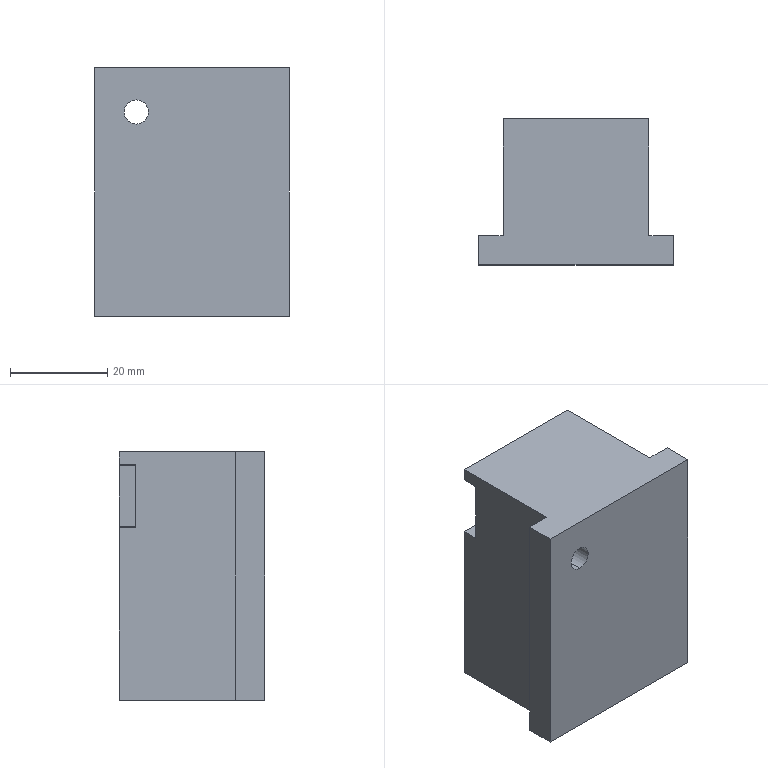Component | SolidWorks | PusherSeat-1 | 1 solid | 23 faces | box 40 x 30 x 51.1 mm | volume 47655 mm3 | plane 14 | cylinder 7 | cone 2 | commonest cylinder face diameters 0.5 x3 5 x2 2.5 x2 | material 201 Annealed Stainless Steel (SS)
build123d program:
from build123d import *

# Parameters (mm, degrees)
SKETCH1_W                 = 40
SKETCH1_H                 = 30
EXTRUDE1_DEPTH            = 30
M3X0_5_TAPPED_HOLE2_D     = 2.5
M3X0_5_TAPPED_HOLE2_DEPTH = 7.5
M3X0_5_TAPPED_HOLE2_TIP   = 0.7511
SKETCH15_W                = 30
SKETCH15_H                = 30
CUT_EXTRUDE5_DEPTH        = 1.2
SKETCH17_3_W              = 6
SKETCH17_3_H              = 5
BOSS_EXTRUDE5_DEPTH       = 30
SKETCH17_3_2_W            = 6
SKETCH17_3_2_H            = 5
BOSS_EXTRUDE6_DEPTH       = 38.8
SKETCH23_W                = 30
SKETCH23_H                = 10
BOSS_EXTRUDE7_DEPTH       = 5
BOSS_EXTRUDE8_DEPTH       = 12.3
SKETCH30_W                = 13
SKETCH30_H                = 19
CUT_EXTRUDE6_DEPTH        = 3.4
SKETCH31_W                = 7.3
SKETCH31_H                = 10
BOSS_EXTRUDE9_DEPTH       = 26.6
SKETCH32_W                = 2.6
SKETCH32_H                = 10
BOSS_EXTRUDE10_DEPTH      = 3.4
SKETCH33_R                = 2.5
CUT_EXTRUDE7_DEPTH        = 68.407
SKETCH34_W                = 6
SKETCH34_H                = 5
BOSS_EXTRUDE11_DEPTH      = 21.1
SKETCH35_R                = 0.25
CUT_EXTRUDE8_DEPTH        = 3.4


with BuildPart() as part:
    # Sketch1 → Extrude1 (new body)
    with BuildSketch(Plane.XY):
        with Locations((20, 15)):
            Rectangle(SKETCH1_W, SKETCH1_H)
    extrude(amount=EXTRUDE1_DEPTH)

    # M3x0.5 Tapped Hole2
    with Locations(Plane.ZY):
        with Locations((15, 15)):
            Hole(M3X0_5_TAPPED_HOLE2_D / 2, depth=M3X0_5_TAPPED_HOLE2_DEPTH)
            with Locations((0, 0, -(M3X0_5_TAPPED_HOLE2_DEPTH + M3X0_5_TAPPED_HOLE2_TIP / 2))):  # 118° drill point
                Cone(0, M3X0_5_TAPPED_HOLE2_D / 2, M3X0_5_TAPPED_HOLE2_TIP, mode=Mode.SUBTRACT)

    # Sketch15 → Cut-Extrude5 (cut)
    with BuildSketch(Plane(origin=(40, 0, 0), x_dir=(0, 0, -1), z_dir=(1, 0, 0))):
        with Locations((-15, 15)):
            Rectangle(SKETCH15_W, SKETCH15_H)
    extrude(amount=-CUT_EXTRUDE5_DEPTH, mode=Mode.SUBTRACT)

    # Sketch17_3 → Boss-Extrude5 (add)
    with BuildSketch(Plane.ZY):
        with Locations((3, -2.5)):
            Rectangle(SKETCH17_3_W, SKETCH17_3_H)
    extrude(amount=-BOSS_EXTRUDE5_DEPTH)

    # Sketch17_3 2 → Boss-Extrude6 (add)
    with BuildSketch(Plane.ZY):
        with Locations((3, 32.5)):
            Rectangle(SKETCH17_3_2_W, SKETCH17_3_2_H)
    extrude(amount=-BOSS_EXTRUDE6_DEPTH)

    # Sketch23 → Boss-Extrude7 (add)
    with BuildSketch(Plane(origin=(38.8, 0, 0), x_dir=(0, 0, -1), z_dir=(1, 0, 0))):
        with Locations((-15, 5)):
            Rectangle(SKETCH23_W, SKETCH23_H)
    extrude(amount=BOSS_EXTRUDE7_DEPTH)

    # Sketch24 → Boss-Extrude8 (add)
    with BuildSketch(Plane(origin=(38.8, 0, 0), x_dir=(0, 0, -1), z_dir=(1, 0, 0))):
        Polygon((-30, 10), (-30, 30), (-6, 30), (-6, 35), (0, 35), (0, 10), align=None)
    extrude(amount=BOSS_EXTRUDE8_DEPTH)

    # Sketch30 → Cut-Extrude6 (cut)
    with BuildSketch(Plane.XY.offset(30)):
        with Locations((42, 9.5)):
            Rectangle(SKETCH30_W, SKETCH30_H)
    extrude(amount=-CUT_EXTRUDE6_DEPTH, mode=Mode.SUBTRACT)

    # Sketch31 → Boss-Extrude9 (add)
    with BuildSketch(Plane(origin=(0, 0, 0), x_dir=(-1, 0, 0), z_dir=(0, 0, -1))):
        with Locations((-47.45, 5)):
            Rectangle(SKETCH31_W, SKETCH31_H)
    extrude(amount=-BOSS_EXTRUDE9_DEPTH)

    # Sketch32 → Boss-Extrude10 (add)
    with BuildSketch(Plane.XY.offset(26.6)):
        with Locations((49.8, 5)):
            Rectangle(SKETCH32_W, SKETCH32_H)
    extrude(amount=BOSS_EXTRUDE10_DEPTH)

    # Sketch33 → Cut-Extrude7 (cut, through all)
    with BuildSketch(Plane.XY.offset(26.6)):
        with Locations((42, 3.55)):
            Circle(SKETCH33_R)
    extrude(amount=-CUT_EXTRUDE7_DEPTH, mode=Mode.SUBTRACT)

    # Sketch34 → Boss-Extrude11 (add)
    with BuildSketch(Plane(origin=(30, 0, 0), x_dir=(0, 0, -1), z_dir=(1, 0, 0))):
        with Locations((-3, -2.5)):
            Rectangle(SKETCH34_W, SKETCH34_H)
    extrude(amount=BOSS_EXTRUDE11_DEPTH)

    # Sketch35 → Cut-Extrude8 (cut)
    with BuildSketch(Plane.XY.offset(30)):
        with Locations((35.5, 19)):
            Circle(SKETCH35_R)
        with Locations((48.5, 19)):
            Circle(SKETCH35_R)
    extrude(amount=-CUT_EXTRUDE8_DEPTH, mode=Mode.SUBTRACT)


solid = part.part

# Placed as in the assembly
solid = solid.moved(Location((-21.915, 5.195, 76.579), (-90, 0, -90)))
STEP:
#1=COLOUR_RGB('',0.7922,0.8196,0.9333);
#2=FILL_AREA_STYLE_COLOUR('',#1);
#3=FILL_AREA_STYLE('',(#2));
#4=SURFACE_STYLE_FILL_AREA(#3);
#5=SURFACE_SIDE_STYLE('',(#4));
#6=SURFACE_STYLE_USAGE(.BOTH.,#5);
#7=PRESENTATION_STYLE_ASSIGNMENT((#6));
#8=CARTESIAN_POINT('',(-0.1148,1.252,4.915));
#9=VERTEX_POINT('',#8);
#10=CARTESIAN_POINT('',(-0.1148,1.252,4.934));
#11=VERTEX_POINT('',#10);
#12=CARTESIAN_POINT('',(-0.1148,1.252,4.924));
#13=DIRECTION('',(0.,-1.,0.));
#14=DIRECTION('',(0.,0.,1.));
#15=AXIS2_PLACEMENT_3D('',#12,#13,#14);
#16=CIRCLE('',#15,0.009843);
#17=EDGE_CURVE('',#9,#11,#16,.T.);
#18=ORIENTED_EDGE('',*,*,#17,.T.);
#19=CARTESIAN_POINT('',(-0.1148,1.386,4.934));
#20=VERTEX_POINT('',#19);
#21=CARTESIAN_POINT('',(-0.1148,1.224,4.934));
#22=DIRECTION('',(-0.,1.,-0.));
#23=VECTOR('',#22,39.37);
#24=LINE('',#21,#23);
#25=EDGE_CURVE('',#11,#20,#24,.T.);
#26=ORIENTED_EDGE('',*,*,#25,.T.);
#27=CARTESIAN_POINT('',(-0.1148,1.386,4.915));
#28=VERTEX_POINT('',#27);
#29=CARTESIAN_POINT('',(-0.1148,1.386,4.924));
#30=DIRECTION('',(-0.,1.,-0.));
#31=DIRECTION('',(0.,0.,1.));
#32=AXIS2_PLACEMENT_3D('',#29,#30,#31);
#33=CIRCLE('',#32,0.009843);
#34=EDGE_CURVE('',#20,#28,#33,.T.);
#35=ORIENTED_EDGE('',*,*,#34,.T.);
#36=CARTESIAN_POINT('',(-0.1148,1.224,4.915));
#37=DIRECTION('',(-0.,1.,-0.));
#38=VECTOR('',#37,39.37);
#39=LINE('',#36,#38);
#40=EDGE_CURVE('',#9,#28,#39,.T.);
#41=ORIENTED_EDGE('',*,*,#40,.F.);
#42=EDGE_LOOP('',(#18,#26,#35,#41));
#43=FACE_OUTER_BOUND('',#42,.T.);
#44=CARTESIAN_POINT('',(-0.1148,1.224,4.924));
#45=DIRECTION('',(-0.,1.,-0.));
#46=DIRECTION('',(0.,0.,1.));
#47=AXIS2_PLACEMENT_3D('',#44,#45,#46);
#48=CYLINDRICAL_SURFACE('',#47,0.009843);
#49=ADVANCED_FACE('',(#43),#48,.F.);
#50=CARTESIAN_POINT('',(-0.723,0.2045,4.767));
#51=VERTEX_POINT('',#50);
#52=CARTESIAN_POINT('',(-0.723,0.2045,4.57));
#53=VERTEX_POINT('',#52);
#54=CARTESIAN_POINT('',(-0.723,0.2045,4.668));
#55=DIRECTION('',(0.,-1.,0.));
#56=DIRECTION('',(0.,0.,-1.));
#57=AXIS2_PLACEMENT_3D('',#54,#55,#56);
#58=CIRCLE('',#57,0.09843);
#59=EDGE_CURVE('',#51,#53,#58,.T.);
#60=ORIENTED_EDGE('',*,*,#59,.T.);
#61=CARTESIAN_POINT('',(-0.723,1.252,4.57));
#62=VERTEX_POINT('',#61);
#63=CARTESIAN_POINT('',(-0.723,0.2045,4.57));
#64=DIRECTION('',(-0.,1.,-0.));
#65=VECTOR('',#64,39.37);
#66=LINE('',#63,#65);
#67=EDGE_CURVE('',#53,#62,#66,.T.);
#68=ORIENTED_EDGE('',*,*,#67,.T.);
#69=CARTESIAN_POINT('',(-0.723,1.252,4.767));
#70=VERTEX_POINT('',#69);
#71=CARTESIAN_POINT('',(-0.723,1.252,4.668));
#72=DIRECTION('',(-0.,1.,-0.));
#73=DIRECTION('',(0.,0.,1.));
#74=AXIS2_PLACEMENT_3D('',#71,#72,#73);
#75=CIRCLE('',#74,0.09843);
#76=EDGE_CURVE('',#62,#70,#75,.T.);
#77=ORIENTED_EDGE('',*,*,#76,.T.);
#78=CARTESIAN_POINT('',(-0.723,0.2045,4.767));
#79=DIRECTION('',(-0.,1.,-0.));
#80=VECTOR('',#79,39.37);
#81=LINE('',#78,#80);
#82=EDGE_CURVE('',#51,#70,#81,.T.);
#83=ORIENTED_EDGE('',*,*,#82,.F.);
#84=EDGE_LOOP('',(#60,#68,#77,#83));
#85=FACE_OUTER_BOUND('',#84,.T.);
#86=CARTESIAN_POINT('',(-0.723,0.2045,4.668));
#87=DIRECTION('',(-0.,1.,-0.));
#88=DIRECTION('',(0.,0.,1.));
#89=AXIS2_PLACEMENT_3D('',#86,#87,#88);
#90=CYLINDRICAL_SURFACE('',#89,0.09843);
#91=ADVANCED_FACE('',(#85),#90,.F.);
#92=CARTESIAN_POINT('',(-0.2722,0.7459,3.31));
#93=VERTEX_POINT('',#92);
#94=CARTESIAN_POINT('',(-0.2722,0.8443,3.31));
#95=VERTEX_POINT('',#94);
#96=CARTESIAN_POINT('',(-0.2722,0.7951,3.31));
#97=DIRECTION('',(0.,0.,-1.));
#98=DIRECTION('',(0.,1.,0.));
#99=AXIS2_PLACEMENT_3D('',#96,#97,#98);
#100=CIRCLE('',#99,0.04921);
#101=EDGE_CURVE('',#93,#95,#100,.T.);
#102=ORIENTED_EDGE('',*,*,#101,.F.);
#103=CARTESIAN_POINT('',(-0.2722,0.7459,3.015));
#104=VERTEX_POINT('',#103);
#105=CARTESIAN_POINT('',(-0.2722,0.7459,3.015));
#106=DIRECTION('',(0.,0.,-1.));
#107=VECTOR('',#106,39.37);
#108=LINE('',#105,#107);
#109=EDGE_CURVE('',#93,#104,#108,.T.);
#110=ORIENTED_EDGE('',*,*,#109,.T.);
#111=CARTESIAN_POINT('',(-0.2722,0.8443,3.015));
#112=VERTEX_POINT('',#111);
#113=CARTESIAN_POINT('',(-0.2722,0.7951,3.015));
#114=DIRECTION('',(0.,0.,-1.));
#115=DIRECTION('',(0.,1.,0.));
#116=AXIS2_PLACEMENT_3D('',#113,#114,#115);
#117=CIRCLE('',#116,0.04921);
#118=EDGE_CURVE('',#104,#112,#117,.T.);
#119=ORIENTED_EDGE('',*,*,#118,.T.);
#120=CARTESIAN_POINT('',(-0.2722,0.8443,3.015));
#121=DIRECTION('',(0.,0.,-1.));
#122=VECTOR('',#121,39.37);
#123=LINE('',#120,#122);
#124=EDGE_CURVE('',#95,#112,#123,.T.);
#125=ORIENTED_EDGE('',*,*,#124,.F.);
#126=EDGE_LOOP('',(#102,#110,#119,#125));
#127=FACE_OUTER_BOUND('',#126,.T.);
#128=CARTESIAN_POINT('',(-0.2722,0.7951,3.015));
#129=DIRECTION('',(0.,0.,-1.));
#130=DIRECTION('',(0.,1.,0.));
#131=AXIS2_PLACEMENT_3D('',#128,#129,#130);
#132=CYLINDRICAL_SURFACE('',#131,0.04921);
#133=ADVANCED_FACE('',(#127),#132,.F.);
#134=CARTESIAN_POINT('',(-0.2722,0.7951,3.34));
#135=VERTEX_POINT('',#134);
#136=CARTESIAN_POINT('',(-0.2722,0.8443,3.31));
#137=DIRECTION('',(0.,0.8572,-0.515));
#138=VECTOR('',#137,39.37);
#139=LINE('',#136,#138);
#140=EDGE_CURVE('',#135,#95,#139,.T.);
#141=ORIENTED_EDGE('',*,*,#140,.F.);
#142=CARTESIAN_POINT('',(-0.2722,0.7459,3.31));
#143=DIRECTION('',(0.,-0.8572,-0.515));
#144=VECTOR('',#143,39.37);
#145=LINE('',#142,#144);
#146=EDGE_CURVE('',#135,#93,#145,.T.);
#147=ORIENTED_EDGE('',*,*,#146,.T.);
#148=ORIENTED_EDGE('',*,*,#101,.T.);
#149=EDGE_LOOP('',(#141,#147,#148));
#150=FACE_OUTER_BOUND('',#149,.T.);
#151=CARTESIAN_POINT('',(-0.2722,0.7951,3.31));
#152=DIRECTION('',(0.,0.,-1.));
#153=DIRECTION('',(0.,1.,0.));
#154=AXIS2_PLACEMENT_3D('',#151,#152,#153);
#155=CONICAL_SURFACE('',#154,0.04921,1.03);
#156=ADVANCED_FACE('',(#150),#155,.F.);
#157=CARTESIAN_POINT('',(-0.8628,0.4407,5.027));
#158=VERTEX_POINT('',#157);
#159=CARTESIAN_POINT('',(-0.8628,0.4407,3.015));
#160=VERTEX_POINT('',#159);
#161=CARTESIAN_POINT('',(-0.8628,0.4407,4.196));
#162=DIRECTION('',(0.,0.,-1.));
#163=VECTOR('',#162,39.37);
#164=LINE('',#161,#163);
#165=EDGE_CURVE('',#158,#160,#164,.T.);
#166=ORIENTED_EDGE('',*,*,#165,.F.);
#167=CARTESIAN_POINT('',(-0.8628,1.386,5.027));
#168=VERTEX_POINT('',#167);
#169=CARTESIAN_POINT('',(-0.8628,1.739,5.027));
#170=DIRECTION('',(0.,-1.,0.));
#171=VECTOR('',#170,39.37);
#172=LINE('',#169,#171);
#173=EDGE_CURVE('',#168,#158,#172,.T.);
#174=ORIENTED_EDGE('',*,*,#173,.F.);
#175=CARTESIAN_POINT('',(-0.8628,1.386,4.924));
#176=VERTEX_POINT('',#175);
#177=CARTESIAN_POINT('',(-0.8628,1.386,4.924));
#178=DIRECTION('',(-0.,-0.,1.));
#179=VECTOR('',#178,39.37);
#180=LINE('',#177,#179);
#181=EDGE_CURVE('',#176,#168,#180,.T.);
#182=ORIENTED_EDGE('',*,*,#181,.F.);
#183=CARTESIAN_POINT('',(-0.8628,1.252,4.924));
#184=VERTEX_POINT('',#183);
#185=CARTESIAN_POINT('',(-0.8628,1.386,4.924));
#186=DIRECTION('',(0.,-1.,0.));
#187=VECTOR('',#186,39.37);
#188=LINE('',#185,#187);
#189=EDGE_CURVE('',#176,#184,#188,.T.);
#190=ORIENTED_EDGE('',*,*,#189,.T.);
#191=CARTESIAN_POINT('',(-0.8628,1.252,4.413));
#192=VERTEX_POINT('',#191);
#193=CARTESIAN_POINT('',(-0.8628,1.252,4.924));
#194=DIRECTION('',(0.,-0.,1.));
#195=VECTOR('',#194,39.37);
#196=LINE('',#193,#195);
#197=EDGE_CURVE('',#192,#184,#196,.T.);
#198=ORIENTED_EDGE('',*,*,#197,.F.);
#199=CARTESIAN_POINT('',(-0.8628,1.386,4.413));
#200=VERTEX_POINT('',#199);
#201=CARTESIAN_POINT('',(-0.8628,1.252,4.413));
#202=DIRECTION('',(-0.,1.,-0.));
#203=VECTOR('',#202,39.37);
#204=LINE('',#201,#203);
#205=EDGE_CURVE('',#192,#200,#204,.T.);
#206=ORIENTED_EDGE('',*,*,#205,.T.);
#207=CARTESIAN_POINT('',(-0.8628,1.386,3.015));
#208=VERTEX_POINT('',#207);
#209=CARTESIAN_POINT('',(-0.8628,1.386,3.015));
#210=DIRECTION('',(-0.,-0.,1.));
#211=VECTOR('',#210,39.37);
#212=LINE('',#209,#211);
#213=EDGE_CURVE('',#208,#200,#212,.T.);
#214=ORIENTED_EDGE('',*,*,#213,.F.);
#215=CARTESIAN_POINT('',(-0.8628,1.386,3.015));
#216=DIRECTION('',(0.,-1.,0.));
#217=VECTOR('',#216,39.37);
#218=LINE('',#215,#217);
#219=EDGE_CURVE('',#208,#160,#218,.T.);
#220=ORIENTED_EDGE('',*,*,#219,.T.);
#221=EDGE_LOOP('',(#166,#174,#182,#190,#198,#206,#214,#220));
#222=FACE_OUTER_BOUND('',#221,.T.);
#223=CARTESIAN_POINT('',(-0.8628,1.386,3.015));
#224=DIRECTION('',(1.,0.,0.));
#225=DIRECTION('',(-0.,1.,-0.));
#226=AXIS2_PLACEMENT_3D('',#223,#224,#225);
#227=PLANE('',#226);
#228=ADVANCED_FACE('',(#222),#227,.F.);
#229=CARTESIAN_POINT('',(-0.1246,1.252,4.924));
#230=VERTEX_POINT('',#229);
#231=CARTESIAN_POINT('',(-0.8628,1.252,4.924));
#232=DIRECTION('',(1.,-0.,0.));
#233=VECTOR('',#232,39.37);
#234=LINE('',#231,#233);
#235=EDGE_CURVE('',#184,#230,#234,.T.);
#236=ORIENTED_EDGE('',*,*,#235,.T.);
#237=CARTESIAN_POINT('',(-0.1148,1.252,4.924));
#238=DIRECTION('',(0.,-1.,0.));
#239=DIRECTION('',(0.,0.,1.));
#240=AXIS2_PLACEMENT_3D('',#237,#238,#239);
#241=CIRCLE('',#240,0.009843);
#242=EDGE_CURVE('',#11,#230,#241,.T.);
#243=ORIENTED_EDGE('',*,*,#242,.F.);
#244=ORIENTED_EDGE('',*,*,#17,.F.);
#245=CARTESIAN_POINT('',(-0.1148,1.252,4.422));
#246=VERTEX_POINT('',#245);
#247=CARTESIAN_POINT('',(-0.1148,1.252,4.924));
#248=DIRECTION('',(-0.,0.,-1.));
#249=VECTOR('',#248,39.37);
#250=LINE('',#247,#249);
#251=EDGE_CURVE('',#9,#246,#250,.T.);
#252=ORIENTED_EDGE('',*,*,#251,.T.);
#253=CARTESIAN_POINT('',(-0.1246,1.252,4.413));
#254=VERTEX_POINT('',#253);
#255=CARTESIAN_POINT('',(-0.1148,1.252,4.413));
#256=DIRECTION('',(0.,-1.,0.));
#257=DIRECTION('',(0.,0.,1.));
#258=AXIS2_PLACEMENT_3D('',#255,#256,#257);
#259=CIRCLE('',#258,0.009843);
#260=EDGE_CURVE('',#254,#246,#259,.T.);
#261=ORIENTED_EDGE('',*,*,#260,.F.);
#262=CARTESIAN_POINT('',(-0.8628,1.252,4.413));
#263=DIRECTION('',(-1.,0.,-0.));
#264=VECTOR('',#263,39.37);
#265=LINE('',#262,#264);
#266=EDGE_CURVE('',#254,#192,#265,.T.);
#267=ORIENTED_EDGE('',*,*,#266,.T.);
#268=ORIENTED_EDGE('',*,*,#197,.T.);
#269=EDGE_LOOP('',(#236,#243,#244,#252,#261,#267,#268));
#270=FACE_OUTER_BOUND('',#269,.T.);
#271=CARTESIAN_POINT('',(-0.723,1.252,4.668));
#272=DIRECTION('',(-0.,1.,-0.));
#273=DIRECTION('',(0.,0.,1.));
#274=AXIS2_PLACEMENT_3D('',#271,#272,#273);
#275=CIRCLE('',#274,0.09843);
#276=EDGE_CURVE('',#70,#62,#275,.T.);
#277=ORIENTED_EDGE('',*,*,#276,.F.);
#278=ORIENTED_EDGE('',*,*,#76,.F.);
#279=EDGE_LOOP('',(#277,#278));
#280=FACE_BOUND('',#279,.T.);
#281=CARTESIAN_POINT('',(-0.8628,1.252,3.015));
#282=DIRECTION('',(-0.,1.,0.));
#283=DIRECTION('',(-0.,-0.,1.));
#284=AXIS2_PLACEMENT_3D('',#281,#282,#283);
#285=PLANE('',#284);
#286=ADVANCED_FACE('',(#270,#280),#285,.T.);
#287=CARTESIAN_POINT('',(0.3183,1.386,5.027));
#288=VERTEX_POINT('',#287);
#289=CARTESIAN_POINT('',(0.3183,1.386,3.015));
#290=VERTEX_POINT('',#289);
#291=CARTESIAN_POINT('',(0.3183,1.386,3.015));
#292=DIRECTION('',(0.,0.,-1.));
#293=VECTOR('',#292,39.37);
#294=LINE('',#291,#293);
#295=EDGE_CURVE('',#288,#290,#294,.T.);
#296=ORIENTED_EDGE('',*,*,#295,.F.);
#297=CARTESIAN_POINT('',(0.3183,0.4407,5.027));
#298=VERTEX_POINT('',#297);
#299=CARTESIAN_POINT('',(0.3183,1.386,5.027));
#300=DIRECTION('',(-0.,1.,-0.));
#301=VECTOR('',#300,39.37);
#302=LINE('',#299,#301);
#303=EDGE_CURVE('',#298,#288,#302,.T.);
#304=ORIENTED_EDGE('',*,*,#303,.F.);
#305=CARTESIAN_POINT('',(0.3183,0.4407,3.015));
#306=VERTEX_POINT('',#305);
#307=CARTESIAN_POINT('',(0.3183,0.4407,4.85));
#308=DIRECTION('',(0.,0.,-1.));
#309=VECTOR('',#308,39.37);
#310=LINE('',#307,#309);
#311=EDGE_CURVE('',#298,#306,#310,.T.);
#312=ORIENTED_EDGE('',*,*,#311,.T.);
#313=CARTESIAN_POINT('',(0.3183,1.386,3.015));
#314=DIRECTION('',(0.,-1.,0.));
#315=VECTOR('',#314,39.37);
#316=LINE('',#313,#315);
#317=EDGE_CURVE('',#290,#306,#316,.T.);
#318=ORIENTED_EDGE('',*,*,#317,.F.);
#319=EDGE_LOOP('',(#296,#304,#312,#318));
#320=FACE_OUTER_BOUND('',#319,.T.);
#321=CARTESIAN_POINT('',(0.3183,1.386,3.015));
#322=DIRECTION('',(-1.,-0.,-0.));
#323=DIRECTION('',(0.,-1.,0.));
#324=AXIS2_PLACEMENT_3D('',#321,#322,#323);
#325=PLANE('',#324);
#326=ADVANCED_FACE('',(#320),#325,.F.);
#327=CARTESIAN_POINT('',(-0.1148,1.386,4.422));
#328=VERTEX_POINT('',#327);
#329=CARTESIAN_POINT('',(-0.1148,1.386,4.924));
#330=DIRECTION('',(-0.,0.,-1.));
#331=VECTOR('',#330,39.37);
#332=LINE('',#329,#331);
#333=EDGE_CURVE('',#28,#328,#332,.T.);
#334=ORIENTED_EDGE('',*,*,#333,.F.);
#335=ORIENTED_EDGE('',*,*,#34,.F.);
#336=CARTESIAN_POINT('',(-0.1246,1.386,4.924));
#337=VERTEX_POINT('',#336);
#338=CARTESIAN_POINT('',(-0.1148,1.386,4.924));
#339=DIRECTION('',(-0.,1.,-0.));
#340=DIRECTION('',(0.,0.,1.));
#341=AXIS2_PLACEMENT_3D('',#338,#339,#340);
#342=CIRCLE('',#341,0.009843);
#343=EDGE_CURVE('',#337,#20,#342,.T.);
#344=ORIENTED_EDGE('',*,*,#343,.F.);
#345=CARTESIAN_POINT('',(-0.8628,1.386,4.924));
#346=DIRECTION('',(1.,-0.,0.));
#347=VECTOR('',#346,39.37);
#348=LINE('',#345,#347);
#349=EDGE_CURVE('',#176,#337,#348,.T.);
#350=ORIENTED_EDGE('',*,*,#349,.F.);
#351=ORIENTED_EDGE('',*,*,#181,.T.);
#352=CARTESIAN_POINT('',(-0.4691,1.386,5.027));
#353=DIRECTION('',(-1.,0.,-0.));
#354=VECTOR('',#353,39.37);
#355=LINE('',#352,#354);
#356=EDGE_CURVE('',#288,#168,#355,.T.);
#357=ORIENTED_EDGE('',*,*,#356,.F.);
#358=ORIENTED_EDGE('',*,*,#295,.T.);
#359=CARTESIAN_POINT('',(-0.8628,1.386,3.015));
#360=DIRECTION('',(-1.,0.,-0.));
#361=VECTOR('',#360,39.37);
#362=LINE('',#359,#361);
#363=EDGE_CURVE('',#290,#208,#362,.T.);
#364=ORIENTED_EDGE('',*,*,#363,.T.);
#365=ORIENTED_EDGE('',*,*,#213,.T.);
#366=CARTESIAN_POINT('',(-0.1246,1.386,4.413));
#367=VERTEX_POINT('',#366);
#368=CARTESIAN_POINT('',(-0.8628,1.386,4.413));
#369=DIRECTION('',(-1.,0.,-0.));
#370=VECTOR('',#369,39.37);
#371=LINE('',#368,#370);
#372=EDGE_CURVE('',#367,#200,#371,.T.);
#373=ORIENTED_EDGE('',*,*,#372,.F.);
#374=CARTESIAN_POINT('',(-0.1148,1.386,4.413));
#375=DIRECTION('',(-0.,1.,-0.));
#376=DIRECTION('',(0.,0.,1.));
#377=AXIS2_PLACEMENT_3D('',#374,#375,#376);
#378=CIRCLE('',#377,0.009843);
#379=EDGE_CURVE('',#328,#367,#378,.T.);
#380=ORIENTED_EDGE('',*,*,#379,.F.);
#381=EDGE_LOOP('',(#334,#335,#344,#350,#351,#357,#358,#364,#365,#373,#380));
#382=FACE_OUTER_BOUND('',#381,.T.);
#383=CARTESIAN_POINT('',(0.3183,1.386,3.015));
#384=DIRECTION('',(0.,-1.,-0.));
#385=DIRECTION('',(0.,0.,-1.));
#386=AXIS2_PLACEMENT_3D('',#383,#384,#385);
#387=PLANE('',#386);
#388=ADVANCED_FACE('',(#382),#387,.F.);
#389=CARTESIAN_POINT('',(-1.06,0.2045,5.027));
#390=VERTEX_POINT('',#389);
#391=CARTESIAN_POINT('',(0.5152,0.2045,5.027));
#392=VERTEX_POINT('',#391);
#393=CARTESIAN_POINT('',(0.5152,0.2045,5.027));
#394=DIRECTION('',(1.,-0.,0.));
#395=VECTOR('',#394,39.37);
#396=LINE('',#393,#395);
#397=EDGE_CURVE('',#390,#392,#396,.T.);
#398=ORIENTED_EDGE('',*,*,#397,.F.);
#399=CARTESIAN_POINT('',(-1.06,0.2045,3.015));
#400=VERTEX_POINT('',#399);
#401=CARTESIAN_POINT('',(-1.06,0.2045,4.196));
#402=DIRECTION('',(0.,0.,-1.));
#403=VECTOR('',#402,39.37);
#404=LINE('',#401,#403);
#405=EDGE_CURVE('',#390,#400,#404,.T.);
#406=ORIENTED_EDGE('',*,*,#405,.T.);
#407=CARTESIAN_POINT('',(0.5152,0.2045,3.015));
#408=VERTEX_POINT('',#407);
#409=CARTESIAN_POINT('',(-0.8628,0.2045,3.015));
#410=DIRECTION('',(-1.,0.,-0.));
#411=VECTOR('',#410,39.37);
#412=LINE('',#409,#411);
#413=EDGE_CURVE('',#408,#400,#412,.T.);
#414=ORIENTED_EDGE('',*,*,#413,.F.);
#415=CARTESIAN_POINT('',(0.5152,0.2045,4.85));
#416=DIRECTION('',(0.,0.,-1.));
#417=VECTOR('',#416,39.37);
#418=LINE('',#415,#417);
#419=EDGE_CURVE('',#392,#408,#418,.T.);
#420=ORIENTED_EDGE('',*,*,#419,.F.);
#421=EDGE_LOOP('',(#398,#406,#414,#420));
#422=FACE_OUTER_BOUND('',#421,.T.);
#423=ORIENTED_EDGE('',*,*,#59,.F.);
#424=CARTESIAN_POINT('',(-0.723,0.2045,4.668));
#425=DIRECTION('',(0.,-1.,0.));
#426=DIRECTION('',(0.,0.,-1.));
#427=AXIS2_PLACEMENT_3D('',#424,#425,#426);
#428=CIRCLE('',#427,0.09843);
#429=EDGE_CURVE('',#53,#51,#428,.T.);
#430=ORIENTED_EDGE('',*,*,#429,.F.);
#431=EDGE_LOOP('',(#423,#430));
#432=FACE_BOUND('',#431,.T.);
#433=CARTESIAN_POINT('',(0.3183,0.2045,3.015));
#434=DIRECTION('',(0.,-1.,-0.));
#435=DIRECTION('',(0.,0.,-1.));
#436=AXIS2_PLACEMENT_3D('',#433,#434,#435);
#437=PLANE('',#436);
#438=ADVANCED_FACE('',(#422,#432),#437,.T.);
#439=CARTESIAN_POINT('',(-0.2722,0.7951,3.015));
#440=DIRECTION('',(0.,0.,-1.));
#441=DIRECTION('',(0.,1.,0.));
#442=AXIS2_PLACEMENT_3D('',#439,#440,#441);
#443=CIRCLE('',#442,0.04921);
#444=EDGE_CURVE('',#112,#104,#443,.T.);
#445=ORIENTED_EDGE('',*,*,#444,.F.);
#446=ORIENTED_EDGE('',*,*,#118,.F.);
#447=EDGE_LOOP('',(#445,#446));
#448=FACE_BOUND('',#447,.T.);
#449=ORIENTED_EDGE('',*,*,#413,.T.);
#450=CARTESIAN_POINT('',(-1.06,0.4407,3.015));
#451=VERTEX_POINT('',#450);
#452=CARTESIAN_POINT('',(-1.06,0.2045,3.015));
#453=DIRECTION('',(-0.,1.,-0.));
#454=VECTOR('',#453,39.37);
#455=LINE('',#452,#454);
#456=EDGE_CURVE('',#400,#451,#455,.T.);
#457=ORIENTED_EDGE('',*,*,#456,.T.);
#458=CARTESIAN_POINT('',(-0.8628,0.4407,3.015));
#459=DIRECTION('',(-1.,0.,-0.));
#460=VECTOR('',#459,39.37);
#461=LINE('',#458,#460);
#462=EDGE_CURVE('',#160,#451,#461,.T.);
#463=ORIENTED_EDGE('',*,*,#462,.F.);
#464=ORIENTED_EDGE('',*,*,#219,.F.);
#465=ORIENTED_EDGE('',*,*,#363,.F.);
#466=ORIENTED_EDGE('',*,*,#317,.T.);
#467=CARTESIAN_POINT('',(0.5152,0.4407,3.015));
#468=VERTEX_POINT('',#467);
#469=CARTESIAN_POINT('',(0.3183,0.4407,3.015));
#470=DIRECTION('',(1.,-0.,0.));
#471=VECTOR('',#470,39.37);
#472=LINE('',#469,#471);
#473=EDGE_CURVE('',#306,#468,#472,.T.);
#474=ORIENTED_EDGE('',*,*,#473,.T.);
#475=CARTESIAN_POINT('',(0.5152,0.2045,3.015));
#476=DIRECTION('',(-0.,1.,-0.));
#477=VECTOR('',#476,39.37);
#478=LINE('',#475,#477);
#479=EDGE_CURVE('',#408,#468,#478,.T.);
#480=ORIENTED_EDGE('',*,*,#479,.F.);
#481=EDGE_LOOP('',(#449,#457,#463,#464,#465,#466,#474,#480));
#482=FACE_OUTER_BOUND('',#481,.T.);
#483=CARTESIAN_POINT('',(-0.8628,1.386,3.015));
#484=DIRECTION('',(-0.,0.,1.));
#485=DIRECTION('',(0.,-1.,0.));
#486=AXIS2_PLACEMENT_3D('',#483,#484,#485);
#487=PLANE('',#486);
#488=ADVANCED_FACE('',(#448,#482),#487,.F.);
#489=ORIENTED_EDGE('',*,*,#146,.F.);
#490=ORIENTED_EDGE('',*,*,#140,.T.);
#491=CARTESIAN_POINT('',(-0.2722,0.7951,3.31));
#492=DIRECTION('',(0.,0.,-1.));
#493=DIRECTION('',(0.,1.,0.));
#494=AXIS2_PLACEMENT_3D('',#491,#492,#493);
#495=CIRCLE('',#494,0.04921);
#496=EDGE_CURVE('',#95,#93,#495,.T.);
#497=ORIENTED_EDGE('',*,*,#496,.T.);
#498=EDGE_LOOP('',(#489,#490,#497));
#499=FACE_OUTER_BOUND('',#498,.T.);
#500=CARTESIAN_POINT('',(-0.2722,0.7951,3.31));
#501=DIRECTION('',(0.,0.,-1.));
#502=DIRECTION('',(0.,1.,0.));
#503=AXIS2_PLACEMENT_3D('',#500,#501,#502);
#504=CONICAL_SURFACE('',#503,0.04921,1.03);
#505=ADVANCED_FACE('',(#499),#504,.F.);
#506=ORIENTED_EDGE('',*,*,#109,.F.);
#507=ORIENTED_EDGE('',*,*,#496,.F.);
#508=ORIENTED_EDGE('',*,*,#124,.T.);
#509=ORIENTED_EDGE('',*,*,#444,.T.);
#510=EDGE_LOOP('',(#506,#507,#508,#509));
#511=FACE_OUTER_BOUND('',#510,.T.);
#512=CARTESIAN_POINT('',(-0.2722,0.7951,3.015));
#513=DIRECTION('',(0.,0.,-1.));
#514=DIRECTION('',(0.,1.,0.));
#515=AXIS2_PLACEMENT_3D('',#512,#513,#514);
#516=CYLINDRICAL_SURFACE('',#515,0.04921);
#517=ADVANCED_FACE('',(#511),#516,.F.);
#518=ORIENTED_EDGE('',*,*,#462,.T.);
#519=CARTESIAN_POINT('',(-1.06,0.4407,5.027));
#520=VERTEX_POINT('',#519);
#521=CARTESIAN_POINT('',(-1.06,0.4407,4.196));
#522=DIRECTION('',(0.,0.,-1.));
#523=VECTOR('',#522,39.37);
#524=LINE('',#521,#523);
#525=EDGE_CURVE('',#520,#451,#524,.T.);
#526=ORIENTED_EDGE('',*,*,#525,.F.);
#527=CARTESIAN_POINT('',(-0.8628,0.4407,5.027));
#528=DIRECTION('',(1.,-0.,0.));
#529=VECTOR('',#528,39.37);
#530=LINE('',#527,#529);
#531=EDGE_CURVE('',#520,#158,#530,.T.);
#532=ORIENTED_EDGE('',*,*,#531,.T.);
#533=ORIENTED_EDGE('',*,*,#165,.T.);
#534=EDGE_LOOP('',(#518,#526,#532,#533));
#535=FACE_OUTER_BOUND('',#534,.T.);
#536=CARTESIAN_POINT('',(-0.8628,0.4407,4.196));
#537=DIRECTION('',(0.,-1.,-0.));
#538=DIRECTION('',(0.,0.,-1.));
#539=AXIS2_PLACEMENT_3D('',#536,#537,#538);
#540=PLANE('',#539);
#541=ADVANCED_FACE('',(#535),#540,.F.);
#542=ORIENTED_EDGE('',*,*,#456,.F.);
#543=ORIENTED_EDGE('',*,*,#405,.F.);
#544=CARTESIAN_POINT('',(-1.06,0.4407,5.027));
#545=DIRECTION('',(-0.,1.,-0.));
#546=VECTOR('',#545,39.37);
#547=LINE('',#544,#546);
#548=EDGE_CURVE('',#390,#520,#547,.T.);
#549=ORIENTED_EDGE('',*,*,#548,.T.);
#550=ORIENTED_EDGE('',*,*,#525,.T.);
#551=EDGE_LOOP('',(#542,#543,#549,#550));
#552=FACE_OUTER_BOUND('',#551,.T.);
#553=CARTESIAN_POINT('',(-1.06,0.2045,4.196));
#554=DIRECTION('',(-1.,-0.,-0.));
#555=DIRECTION('',(0.,-1.,0.));
#556=AXIS2_PLACEMENT_3D('',#553,#554,#555);
#557=PLANE('',#556);
#558=ADVANCED_FACE('',(#552),#557,.T.);
#559=ORIENTED_EDGE('',*,*,#311,.F.);
#560=CARTESIAN_POINT('',(0.5152,0.4407,5.027));
#561=VERTEX_POINT('',#560);
#562=CARTESIAN_POINT('',(0.3183,0.4407,5.027));
#563=DIRECTION('',(-1.,0.,-0.));
#564=VECTOR('',#563,39.37);
#565=LINE('',#562,#564);
#566=EDGE_CURVE('',#561,#298,#565,.T.);
#567=ORIENTED_EDGE('',*,*,#566,.F.);
#568=CARTESIAN_POINT('',(0.5152,0.4407,4.85));
#569=DIRECTION('',(0.,0.,-1.));
#570=VECTOR('',#569,39.37);
#571=LINE('',#568,#570);
#572=EDGE_CURVE('',#561,#468,#571,.T.);
#573=ORIENTED_EDGE('',*,*,#572,.T.);
#574=ORIENTED_EDGE('',*,*,#473,.F.);
#575=EDGE_LOOP('',(#559,#567,#573,#574));
#576=FACE_OUTER_BOUND('',#575,.T.);
#577=CARTESIAN_POINT('',(0.3183,0.4407,4.85));
#578=DIRECTION('',(-0.,1.,0.));
#579=DIRECTION('',(-0.,-0.,1.));
#580=AXIS2_PLACEMENT_3D('',#577,#578,#579);
#581=PLANE('',#580);
#582=ADVANCED_FACE('',(#576),#581,.T.);
#583=ORIENTED_EDGE('',*,*,#572,.F.);
#584=CARTESIAN_POINT('',(0.5152,0.4407,5.027));
#585=DIRECTION('',(-0.,1.,-0.));
#586=VECTOR('',#585,39.37);
#587=LINE('',#584,#586);
#588=EDGE_CURVE('',#392,#561,#587,.T.);
#589=ORIENTED_EDGE('',*,*,#588,.F.);
#590=ORIENTED_EDGE('',*,*,#419,.T.);
#591=ORIENTED_EDGE('',*,*,#479,.T.);
#592=EDGE_LOOP('',(#583,#589,#590,#591));
#593=FACE_OUTER_BOUND('',#592,.T.);
#594=CARTESIAN_POINT('',(0.5152,0.2045,4.85));
#595=DIRECTION('',(-1.,-0.,-0.));
#596=DIRECTION('',(0.,-1.,0.));
#597=AXIS2_PLACEMENT_3D('',#594,#595,#596);
#598=PLANE('',#597);
#599=ADVANCED_FACE('',(#593),#598,.F.);
#600=ORIENTED_EDGE('',*,*,#356,.T.);
#601=ORIENTED_EDGE('',*,*,#173,.T.);
#602=ORIENTED_EDGE('',*,*,#531,.F.);
#603=ORIENTED_EDGE('',*,*,#548,.F.);
#604=ORIENTED_EDGE('',*,*,#397,.T.);
#605=ORIENTED_EDGE('',*,*,#588,.T.);
#606=ORIENTED_EDGE('',*,*,#566,.T.);
#607=ORIENTED_EDGE('',*,*,#303,.T.);
#608=EDGE_LOOP('',(#600,#601,#602,#603,#604,#605,#606,#607));
#609=FACE_OUTER_BOUND('',#608,.T.);
#610=CARTESIAN_POINT('',(-0.8628,0.2045,5.027));
#611=DIRECTION('',(0.,-0.,-1.));
#612=DIRECTION('',(-0.,1.,-0.));
#613=AXIS2_PLACEMENT_3D('',#610,#611,#612);
#614=PLANE('',#613);
#615=ADVANCED_FACE('',(#609),#614,.F.);
#616=ORIENTED_EDGE('',*,*,#349,.T.);
#617=CARTESIAN_POINT('',(-0.1246,1.224,4.924));
#618=DIRECTION('',(0.,-1.,0.));
#619=VECTOR('',#618,39.37);
#620=LINE('',#617,#619);
#621=EDGE_CURVE('',#337,#230,#620,.T.);
#622=ORIENTED_EDGE('',*,*,#621,.T.);
#623=ORIENTED_EDGE('',*,*,#235,.F.);
#624=ORIENTED_EDGE('',*,*,#189,.F.);
#625=EDGE_LOOP('',(#616,#622,#623,#624));
#626=FACE_OUTER_BOUND('',#625,.T.);
#627=CARTESIAN_POINT('',(-0.8628,1.252,4.924));
#628=DIRECTION('',(-0.,0.,1.));
#629=DIRECTION('',(0.,-1.,0.));
#630=AXIS2_PLACEMENT_3D('',#627,#628,#629);
#631=PLANE('',#630);
#632=ADVANCED_FACE('',(#626),#631,.F.);
#633=ORIENTED_EDGE('',*,*,#266,.F.);
#634=CARTESIAN_POINT('',(-0.1246,1.224,4.413));
#635=DIRECTION('',(-0.,1.,-0.));
#636=VECTOR('',#635,39.37);
#637=LINE('',#634,#636);
#638=EDGE_CURVE('',#254,#367,#637,.T.);
#639=ORIENTED_EDGE('',*,*,#638,.T.);
#640=ORIENTED_EDGE('',*,*,#372,.T.);
#641=ORIENTED_EDGE('',*,*,#205,.F.);
#642=EDGE_LOOP('',(#633,#639,#640,#641));
#643=FACE_OUTER_BOUND('',#642,.T.);
#644=CARTESIAN_POINT('',(-0.8628,1.252,4.413));
#645=DIRECTION('',(0.,-0.,-1.));
#646=DIRECTION('',(-0.,1.,-0.));
#647=AXIS2_PLACEMENT_3D('',#644,#645,#646);
#648=PLANE('',#647);
#649=ADVANCED_FACE('',(#643),#648,.F.);
#650=ORIENTED_EDGE('',*,*,#251,.F.);
#651=ORIENTED_EDGE('',*,*,#40,.T.);
#652=ORIENTED_EDGE('',*,*,#333,.T.);
#653=CARTESIAN_POINT('',(-0.1148,1.224,4.422));
#654=DIRECTION('',(0.,-1.,0.));
#655=VECTOR('',#654,39.37);
#656=LINE('',#653,#655);
#657=EDGE_CURVE('',#328,#246,#656,.T.);
#658=ORIENTED_EDGE('',*,*,#657,.T.);
#659=EDGE_LOOP('',(#650,#651,#652,#658));
#660=FACE_OUTER_BOUND('',#659,.T.);
#661=CARTESIAN_POINT('',(-0.1148,1.252,4.924));
#662=DIRECTION('',(1.,-0.,-0.));
#663=DIRECTION('',(-0.,0.,-1.));
#664=AXIS2_PLACEMENT_3D('',#661,#662,#663);
#665=PLANE('',#664);
#666=ADVANCED_FACE('',(#660),#665,.F.);
#667=ORIENTED_EDGE('',*,*,#67,.F.);
#668=ORIENTED_EDGE('',*,*,#429,.T.);
#669=ORIENTED_EDGE('',*,*,#82,.T.);
#670=ORIENTED_EDGE('',*,*,#276,.T.);
#671=EDGE_LOOP('',(#667,#668,#669,#670));
#672=FACE_OUTER_BOUND('',#671,.T.);
#673=CARTESIAN_POINT('',(-0.723,0.2045,4.668));
#674=DIRECTION('',(-0.,1.,-0.));
#675=DIRECTION('',(0.,0.,1.));
#676=AXIS2_PLACEMENT_3D('',#673,#674,#675);
#677=CYLINDRICAL_SURFACE('',#676,0.09843);
#678=ADVANCED_FACE('',(#672),#677,.F.);
#679=ORIENTED_EDGE('',*,*,#260,.T.);
#680=ORIENTED_EDGE('',*,*,#657,.F.);
#681=ORIENTED_EDGE('',*,*,#379,.T.);
#682=ORIENTED_EDGE('',*,*,#638,.F.);
#683=EDGE_LOOP('',(#679,#680,#681,#682));
#684=FACE_OUTER_BOUND('',#683,.T.);
#685=CARTESIAN_POINT('',(-0.1148,1.224,4.413));
#686=DIRECTION('',(-0.,1.,-0.));
#687=DIRECTION('',(0.,0.,1.));
#688=AXIS2_PLACEMENT_3D('',#685,#686,#687);
#689=CYLINDRICAL_SURFACE('',#688,0.009843);
#690=ADVANCED_FACE('',(#684),#689,.F.);
#691=ORIENTED_EDGE('',*,*,#25,.F.);
#692=ORIENTED_EDGE('',*,*,#242,.T.);
#693=ORIENTED_EDGE('',*,*,#621,.F.);
#694=ORIENTED_EDGE('',*,*,#343,.T.);
#695=EDGE_LOOP('',(#691,#692,#693,#694));
#696=FACE_OUTER_BOUND('',#695,.T.);
#697=CARTESIAN_POINT('',(-0.1148,1.224,4.924));
#698=DIRECTION('',(-0.,1.,-0.));
#699=DIRECTION('',(0.,0.,1.));
#700=AXIS2_PLACEMENT_3D('',#697,#698,#699);
#701=CYLINDRICAL_SURFACE('',#700,0.009843);
#702=ADVANCED_FACE('',(#696),#701,.F.);
#703=CLOSED_SHELL('',(#49,#91,#133,#156,#228,#286,#326,#388,#438,#488,#505,#517,#541,#558,#582,#599,#615,#632,#649,#666,#678,#690,#702));
#704=MANIFOLD_SOLID_BREP('',#703);
#705=STYLED_ITEM('',(#7),#704);
#706=PRESENTATION_LAYER_ASSIGNMENT('','',(#705));
#707=CARTESIAN_POINT('',(0.,0.,0.));
#708=DIRECTION('',(0.,0.,1.));
#709=DIRECTION('',(1.,0.,0.));
#710=AXIS2_PLACEMENT_3D('',#707,#708,#709);
#711=(LENGTH_UNIT()NAMED_UNIT(*)SI_UNIT($,.METRE.));
#712=LENGTH_MEASURE_WITH_UNIT(LENGTH_MEASURE(0.0254),#711);
#713=DIMENSIONAL_EXPONENTS(1.,0.,0.,0.,0.,0.,0.);
#714=(CONVERSION_BASED_UNIT('',#712)LENGTH_UNIT()NAMED_UNIT(#713));
#715=UNCERTAINTY_MEASURE_WITH_UNIT(LENGTH_MEASURE(0.00001),#714,'','');
#716=(NAMED_UNIT(*)PLANE_ANGLE_UNIT()SI_UNIT($,.RADIAN.));
#717=(NAMED_UNIT(*)SI_UNIT($,.STERADIAN.)SOLID_ANGLE_UNIT());
#718=(GEOMETRIC_REPRESENTATION_CONTEXT(3)GLOBAL_UNCERTAINTY_ASSIGNED_CONTEXT((#715))GLOBAL_UNIT_ASSIGNED_CONTEXT((#714,#716,#717))REPRESENTATION_CONTEXT('',''));
#719=ADVANCED_BREP_SHAPE_REPRESENTATION('',(#704,#710),#718);
#720=(LENGTH_UNIT()NAMED_UNIT(*)SI_UNIT($,.METRE.));
#721=LENGTH_MEASURE_WITH_UNIT(LENGTH_MEASURE(0.0254),#720);
#722=DIMENSIONAL_EXPONENTS(1.,0.,0.,0.,0.,0.,0.);
#723=(CONVERSION_BASED_UNIT('',#721)LENGTH_UNIT()NAMED_UNIT(#722));
#724=UNCERTAINTY_MEASURE_WITH_UNIT(LENGTH_MEASURE(0.00001),#723,'','');
#725=(NAMED_UNIT(*)PLANE_ANGLE_UNIT()SI_UNIT($,.RADIAN.));
#726=(NAMED_UNIT(*)SI_UNIT($,.STERADIAN.)SOLID_ANGLE_UNIT());
#727=(GEOMETRIC_REPRESENTATION_CONTEXT(3)GLOBAL_UNCERTAINTY_ASSIGNED_CONTEXT((#724))GLOBAL_UNIT_ASSIGNED_CONTEXT((#723,#725,#726))REPRESENTATION_CONTEXT('',''));
#728=MECHANICAL_DESIGN_GEOMETRIC_PRESENTATION_REPRESENTATION('',(#705),#727);